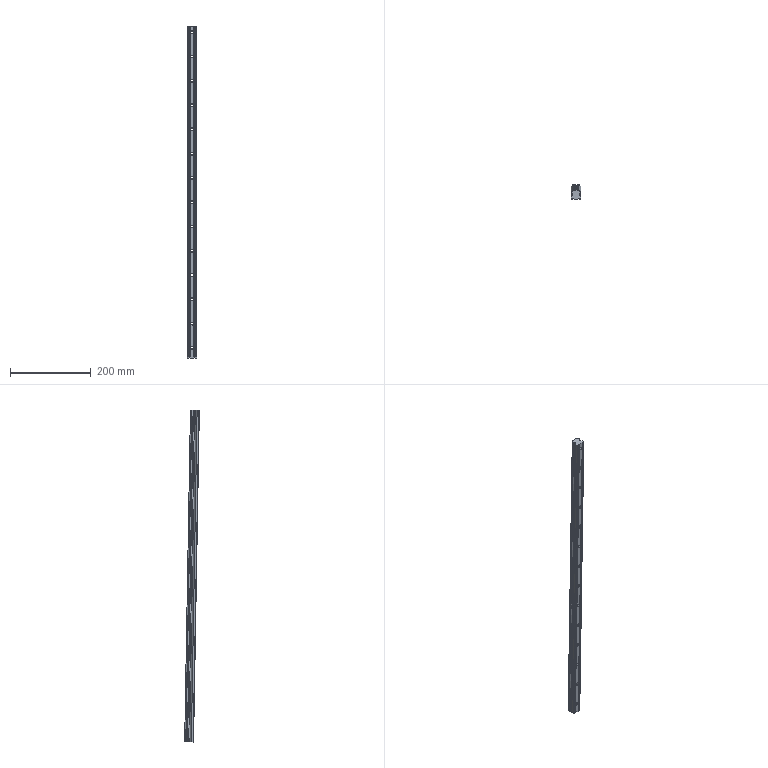Component | SolidWorks | HGH25CAGuideRail(FrontAndRear)-1 | 1 solid | 107 faces | volume 341625 mm3 | cylinder 60 | plane 47 | commonest cylinder face diameters 11 x28 7 x28 4.6 x4